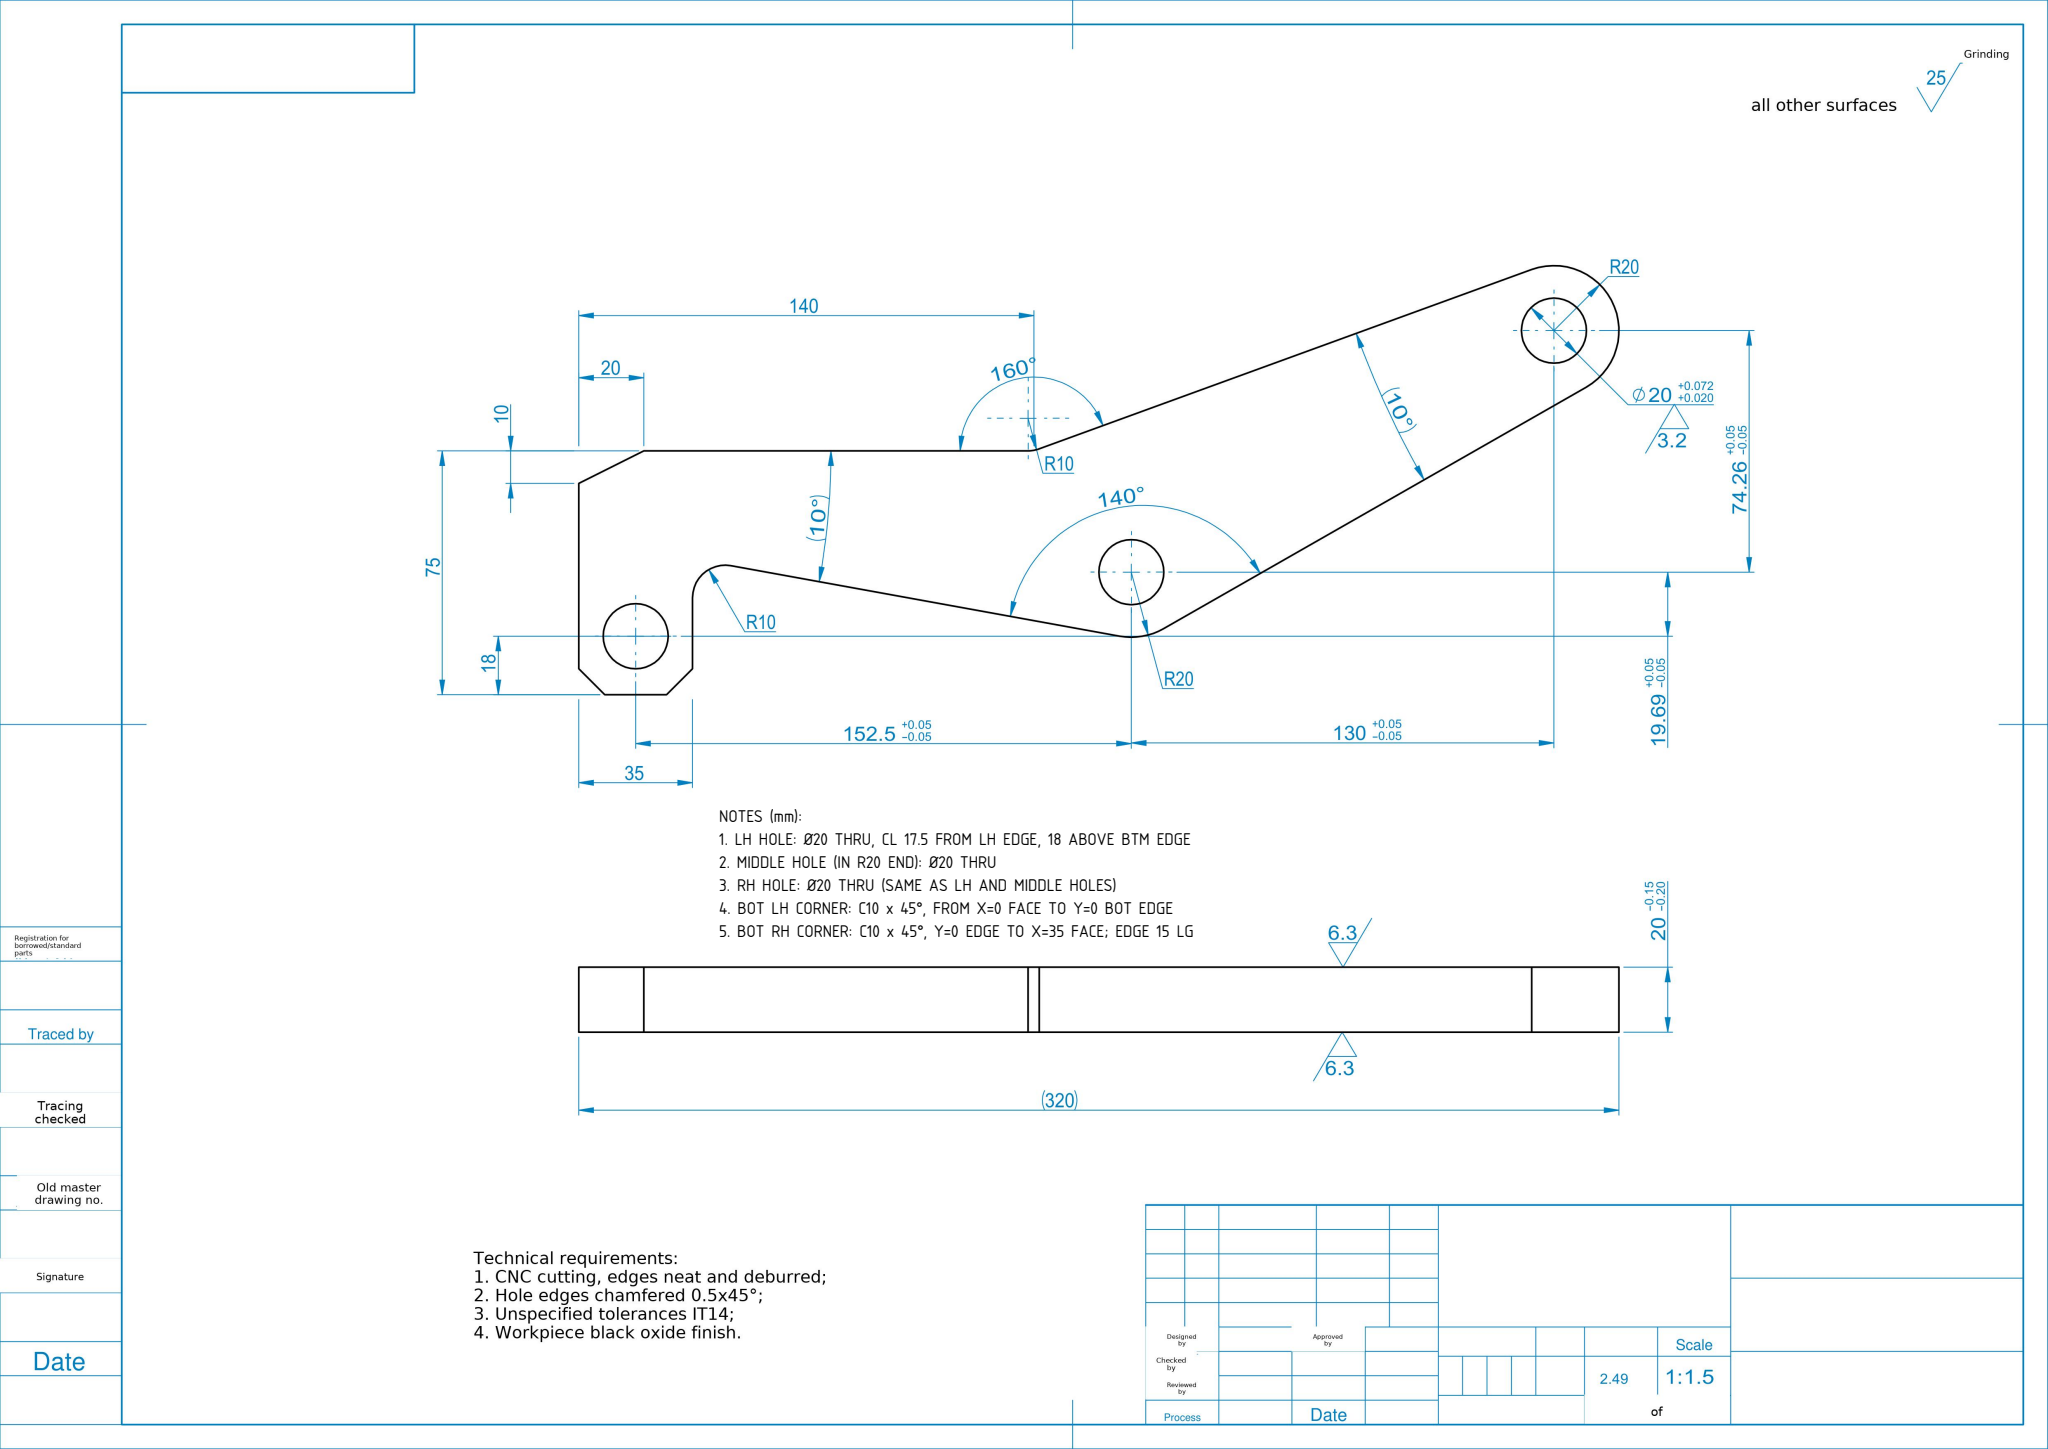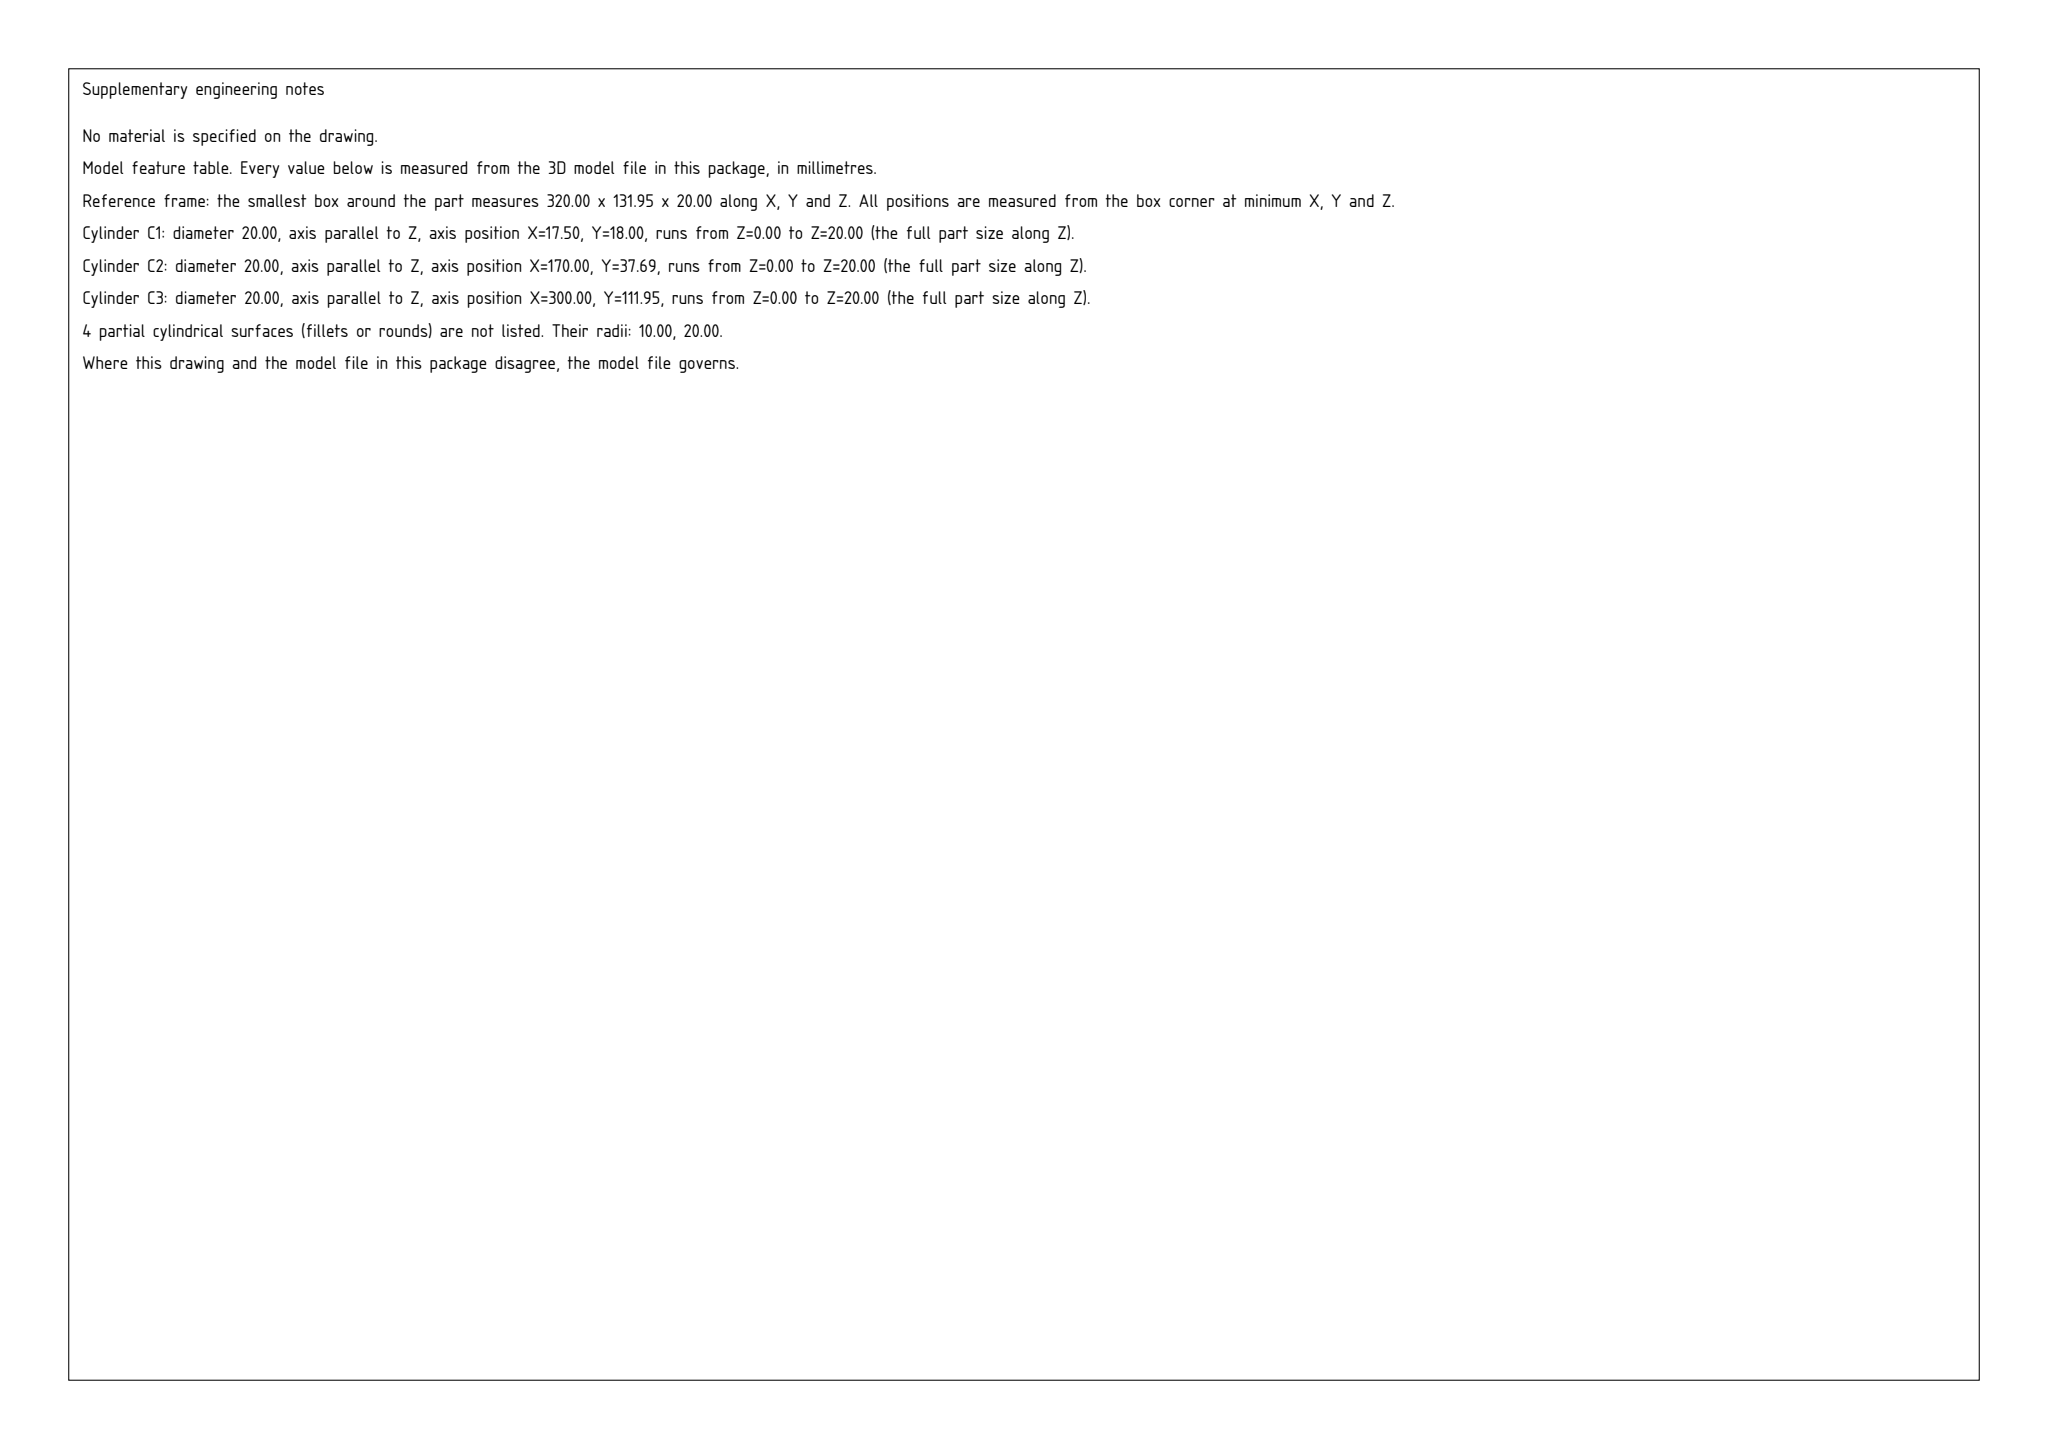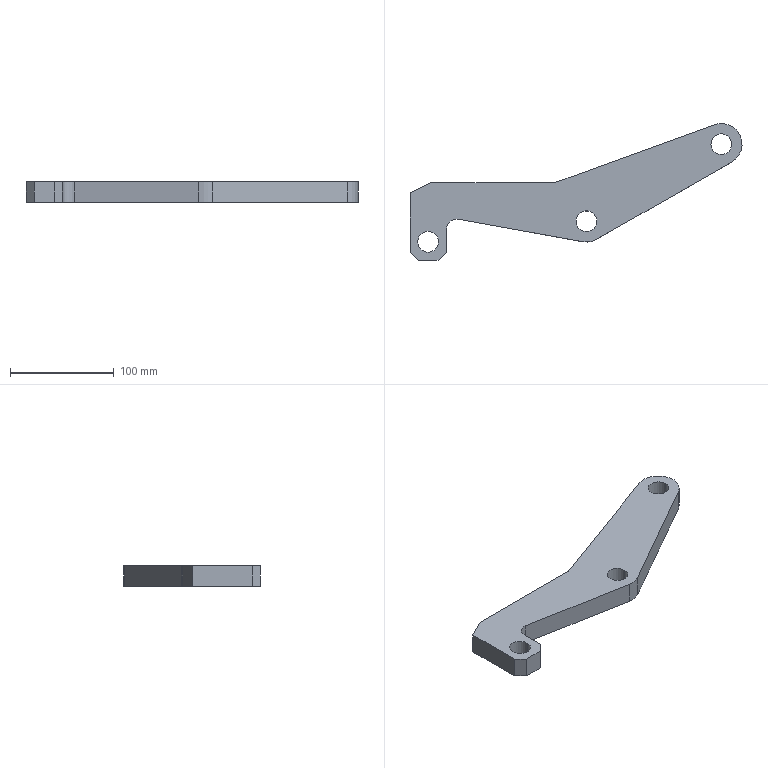Part | SolidWorks | mm | 1 solid | 22 faces | box 320 x 131.95 x 20 mm | volume 319656 mm3 | plane 12 | cylinder 10 | commonest cylinder face diameters 20 x8 40 x2
Drawing notes:
LH HOLE: Ø20 THRU, CL 17.5 FROM LH EDGE, 18 ABOVE BTM EDGE | from the solid: cylinder dia 20.0, axis z, pos (17.5, 18.0), length 20.0 (thru 20 thk)
MIDDLE HOLE (IN R20 END): Ø20 THRU | from the solid: cylinder dia 20.0, axis z, pos (170.0, 37.69), length 20.0, coaxial with 40.0 dia R20 end
RH HOLE: Ø20 THRU (SAME AS LH AND MIDDLE HOLES) | from the solid: cylinder dia 20.0, axis z, pos (300.0, 111.95), coaxial with 40.0 dia R20 end
BOT LH CORNER: C10 x 45°, FROM X=0 FACE TO Y=0 BOT EDGE | from the solid: Planes x=0, y=0 of left block (bbox min corner); chamfer face runs 45° between them, legs 10 x 10, i.e. starts 10 up x=0 face and 10 along y=0 edge
BOT RH CORNER: C10 x 45°, Y=0 EDGE TO X=35 FACE; EDGE 15 LG | from the solid: Planes y=0 and x=35; 45° chamfer legs 10 x 10 -> bottom edge runs x=10 to x=25 (15 lg), x=35 face starts at y=10
build123d program:
from build123d import *

# Parameters (mm, degrees)
BOSS_EXTRUDE1_DEPTH = 10
SKETCH2_R           = 10
CUT_EXTRUDE1_DEPTH  = 347.715
CHAMFER2_SIZE       = 8
CHAMFER3_SIZE       = 20
CHAMFER3_SIZE2      = 10
FILLET1_R           = 10
SKETCH5_R           = 10
CUT_EXTRUDE3_DEPTH  = 347.715
SKETCH7_R           = 10
CUT_EXTRUDE5_DEPTH  = 347.715
CUT_EXTRUDE6_DEPTH  = 347.715
FILLET4_R           = 10


with BuildPart() as part:
    # Sketch1 → Boss-Extrude1 (new, symmetric)
    with BuildSketch(Plane.XY):
        with BuildLine():
            Line((140, 75), (293.16, 130.746))
            ThreePointArc((293.16, 130.746), (318.146, 120.362), (309.92, 94.585))
            Line((309.92, 94.585), (179.92, 20.325))
            ThreePointArc((179.92, 20.325), (173.382, 17.979), (166.436, 18.011))
            Line((166.436, 18.011), (45, 40))
            Line((45, 40), (35, 30))
            Line((35, 30), (35, 0))
            Line((35, 0), (0, 0))
            Line((0, 0), (0, 75))
            Line((0, 75), (140, 75))
        make_face()
    extrude(amount=BOSS_EXTRUDE1_DEPTH, both=True)

    # Sketch2 → Cut-Extrude1 (cut, through all)
    with BuildSketch(Plane.XY.offset(10)):
        with Locations((300, 111.952)):
            Circle(SKETCH2_R)
    extrude(amount=-CUT_EXTRUDE1_DEPTH, mode=Mode.SUBTRACT)

    # Chamfer2
    chamfer2_edges = [part.edges().sort_by_distance(p)[0] for p in [
        (35, 0, 0),
        (0, 0, 0),
    ]]
    chamfer(chamfer2_edges, length=CHAMFER2_SIZE)

    # Chamfer3
    chamfer3_edges = [part.edges().sort_by_distance(p)[0] for p in [
        (0, 75, 0),
    ]]
    chamfer3_side = [part.faces().sort_by_distance(p)[0] for p in [
        (70, 75, 0),
    ]]
    chamfer(chamfer3_edges, length=CHAMFER3_SIZE, length2=CHAMFER3_SIZE2, reference=chamfer3_side[0])

    # Fillet1
    fillet1_edges = [part.edges().sort_by_distance(p)[0] for p in [
        (140, 75, 0),
    ]]
    fillet(fillet1_edges, radius=FILLET1_R)

    # Sketch5 → Cut-Extrude3 (cut, through all)
    with BuildSketch(Plane.XY.offset(10)):
        with Locations((17.5, 18)):
            Circle(SKETCH5_R)
    extrude(amount=-CUT_EXTRUDE3_DEPTH, mode=Mode.SUBTRACT)

    # Sketch7 → Cut-Extrude5 (cut, through all)
    with BuildSketch(Plane.XY.offset(10)):
        with Locations((170, 37.691)):
            Circle(SKETCH7_R)
    extrude(amount=-CUT_EXTRUDE5_DEPTH, mode=Mode.SUBTRACT)

    # Sketch8 → Cut-Extrude6 (cut, through all)
    with BuildSketch(Plane.XY.offset(10)):
        Polygon((35, 30), (35, 41.811), (45, 40), align=None)
    extrude(amount=-CUT_EXTRUDE6_DEPTH, mode=Mode.SUBTRACT)

    # Fillet4
    fillet4_edges = [part.edges().sort_by_distance(p)[0] for p in [
        (35, 41.811, 0),
    ]]
    fillet(fillet4_edges, radius=FILLET4_R)


solid = part.part
STEP:
#1=CARTESIAN_POINT('',(160.,37.691,-10.));
#2=VERTEX_POINT('',#1);
#3=CARTESIAN_POINT('',(180.,37.691,-10.));
#4=VERTEX_POINT('',#3);
#5=CARTESIAN_POINT('',(170.,37.691,-10.));
#6=DIRECTION('',(0.,0.,1.));
#7=DIRECTION('',(1.,0.,0.));
#8=AXIS2_PLACEMENT_3D('',#5,#6,#7);
#9=CIRCLE('',#8,10.);
#10=EDGE_CURVE('',#2,#4,#9,.T.);
#11=ORIENTED_EDGE('',*,*,#10,.F.);
#12=CARTESIAN_POINT('',(160.,37.691,10.));
#13=VERTEX_POINT('',#12);
#14=CARTESIAN_POINT('',(160.,37.691,-10.));
#15=DIRECTION('',(0.,0.,1.));
#16=VECTOR('',#15,1000.);
#17=LINE('',#14,#16);
#18=EDGE_CURVE('',#2,#13,#17,.T.);
#19=ORIENTED_EDGE('',*,*,#18,.T.);
#20=CARTESIAN_POINT('',(180.,37.691,10.));
#21=VERTEX_POINT('',#20);
#22=CARTESIAN_POINT('',(170.,37.691,10.));
#23=DIRECTION('',(0.,0.,1.));
#24=DIRECTION('',(1.,0.,0.));
#25=AXIS2_PLACEMENT_3D('',#22,#23,#24);
#26=CIRCLE('',#25,10.);
#27=EDGE_CURVE('',#13,#21,#26,.T.);
#28=ORIENTED_EDGE('',*,*,#27,.T.);
#29=CARTESIAN_POINT('',(180.,37.691,-10.));
#30=DIRECTION('',(0.,0.,1.));
#31=VECTOR('',#30,1000.);
#32=LINE('',#29,#31);
#33=EDGE_CURVE('',#4,#21,#32,.T.);
#34=ORIENTED_EDGE('',*,*,#33,.F.);
#35=EDGE_LOOP('',(#11,#19,#28,#34));
#36=FACE_OUTER_BOUND('',#35,.T.);
#37=CARTESIAN_POINT('',(170.,37.691,-10.));
#38=DIRECTION('',(0.,0.,1.));
#39=DIRECTION('',(1.,0.,0.));
#40=AXIS2_PLACEMENT_3D('',#37,#38,#39);
#41=CYLINDRICAL_SURFACE('',#40,10.);
#42=ADVANCED_FACE('',(#36),#41,.F.);
#43=CARTESIAN_POINT('',(7.5,18.,-10.));
#44=VERTEX_POINT('',#43);
#45=CARTESIAN_POINT('',(27.5,18.,-10.));
#46=VERTEX_POINT('',#45);
#47=CARTESIAN_POINT('',(17.5,18.,-10.));
#48=DIRECTION('',(0.,0.,1.));
#49=DIRECTION('',(1.,0.,0.));
#50=AXIS2_PLACEMENT_3D('',#47,#48,#49);
#51=CIRCLE('',#50,10.);
#52=EDGE_CURVE('',#44,#46,#51,.T.);
#53=ORIENTED_EDGE('',*,*,#52,.F.);
#54=CARTESIAN_POINT('',(7.5,18.,10.));
#55=VERTEX_POINT('',#54);
#56=CARTESIAN_POINT('',(7.5,18.,-10.));
#57=DIRECTION('',(0.,0.,1.));
#58=VECTOR('',#57,1000.);
#59=LINE('',#56,#58);
#60=EDGE_CURVE('',#44,#55,#59,.T.);
#61=ORIENTED_EDGE('',*,*,#60,.T.);
#62=CARTESIAN_POINT('',(27.5,18.,10.));
#63=VERTEX_POINT('',#62);
#64=CARTESIAN_POINT('',(17.5,18.,10.));
#65=DIRECTION('',(0.,0.,1.));
#66=DIRECTION('',(1.,0.,0.));
#67=AXIS2_PLACEMENT_3D('',#64,#65,#66);
#68=CIRCLE('',#67,10.);
#69=EDGE_CURVE('',#55,#63,#68,.T.);
#70=ORIENTED_EDGE('',*,*,#69,.T.);
#71=CARTESIAN_POINT('',(27.5,18.,-10.));
#72=DIRECTION('',(0.,0.,1.));
#73=VECTOR('',#72,1000.);
#74=LINE('',#71,#73);
#75=EDGE_CURVE('',#46,#63,#74,.T.);
#76=ORIENTED_EDGE('',*,*,#75,.F.);
#77=EDGE_LOOP('',(#53,#61,#70,#76));
#78=FACE_OUTER_BOUND('',#77,.T.);
#79=CARTESIAN_POINT('',(17.5,18.,-10.));
#80=DIRECTION('',(0.,0.,1.));
#81=DIRECTION('',(1.,0.,0.));
#82=AXIS2_PLACEMENT_3D('',#79,#80,#81);
#83=CYLINDRICAL_SURFACE('',#82,10.);
#84=ADVANCED_FACE('',(#78),#83,.F.);
#85=CARTESIAN_POINT('',(290.,111.952,-10.));
#86=VERTEX_POINT('',#85);
#87=CARTESIAN_POINT('',(310.,111.952,-10.));
#88=VERTEX_POINT('',#87);
#89=CARTESIAN_POINT('',(300.,111.952,-10.));
#90=DIRECTION('',(0.,0.,1.));
#91=DIRECTION('',(1.,0.,0.));
#92=AXIS2_PLACEMENT_3D('',#89,#90,#91);
#93=CIRCLE('',#92,10.);
#94=EDGE_CURVE('',#86,#88,#93,.T.);
#95=ORIENTED_EDGE('',*,*,#94,.F.);
#96=CARTESIAN_POINT('',(290.,111.952,10.));
#97=VERTEX_POINT('',#96);
#98=CARTESIAN_POINT('',(290.,111.952,-10.));
#99=DIRECTION('',(0.,0.,1.));
#100=VECTOR('',#99,1000.);
#101=LINE('',#98,#100);
#102=EDGE_CURVE('',#86,#97,#101,.T.);
#103=ORIENTED_EDGE('',*,*,#102,.T.);
#104=CARTESIAN_POINT('',(310.,111.952,10.));
#105=VERTEX_POINT('',#104);
#106=CARTESIAN_POINT('',(300.,111.952,10.));
#107=DIRECTION('',(0.,0.,1.));
#108=DIRECTION('',(1.,0.,0.));
#109=AXIS2_PLACEMENT_3D('',#106,#107,#108);
#110=CIRCLE('',#109,10.);
#111=EDGE_CURVE('',#97,#105,#110,.T.);
#112=ORIENTED_EDGE('',*,*,#111,.T.);
#113=CARTESIAN_POINT('',(310.,111.952,-10.));
#114=DIRECTION('',(0.,0.,1.));
#115=VECTOR('',#114,1000.);
#116=LINE('',#113,#115);
#117=EDGE_CURVE('',#88,#105,#116,.T.);
#118=ORIENTED_EDGE('',*,*,#117,.F.);
#119=EDGE_LOOP('',(#95,#103,#112,#118));
#120=FACE_OUTER_BOUND('',#119,.T.);
#121=CARTESIAN_POINT('',(300.,111.952,-10.));
#122=DIRECTION('',(0.,0.,1.));
#123=DIRECTION('',(1.,0.,0.));
#124=AXIS2_PLACEMENT_3D('',#121,#122,#123);
#125=CYLINDRICAL_SURFACE('',#124,10.);
#126=ADVANCED_FACE('',(#120),#125,.F.);
#127=CARTESIAN_POINT('',(46.782,39.677,10.));
#128=VERTEX_POINT('',#127);
#129=CARTESIAN_POINT('',(166.436,18.011,10.));
#130=VERTEX_POINT('',#129);
#131=CARTESIAN_POINT('',(45.,40.,10.));
#132=DIRECTION('',(0.984,-0.1782,0.));
#133=VECTOR('',#132,1000.);
#134=LINE('',#131,#133);
#135=EDGE_CURVE('',#128,#130,#134,.T.);
#136=ORIENTED_EDGE('',*,*,#135,.F.);
#137=CARTESIAN_POINT('',(46.782,39.677,-10.));
#138=VERTEX_POINT('',#137);
#139=CARTESIAN_POINT('',(46.782,39.677,-10.));
#140=DIRECTION('',(0.,0.,-1.));
#141=VECTOR('',#140,1000.);
#142=LINE('',#139,#141);
#143=EDGE_CURVE('',#128,#138,#142,.T.);
#144=ORIENTED_EDGE('',*,*,#143,.T.);
#145=CARTESIAN_POINT('',(166.436,18.011,-10.));
#146=VERTEX_POINT('',#145);
#147=CARTESIAN_POINT('',(45.,40.,-10.));
#148=DIRECTION('',(0.984,-0.1782,0.));
#149=VECTOR('',#148,1000.);
#150=LINE('',#147,#149);
#151=EDGE_CURVE('',#138,#146,#150,.T.);
#152=ORIENTED_EDGE('',*,*,#151,.T.);
#153=CARTESIAN_POINT('',(166.436,18.011,10.));
#154=DIRECTION('',(0.,0.,-1.));
#155=VECTOR('',#154,1000.);
#156=LINE('',#153,#155);
#157=EDGE_CURVE('',#130,#146,#156,.T.);
#158=ORIENTED_EDGE('',*,*,#157,.F.);
#159=EDGE_LOOP('',(#136,#144,#152,#158));
#160=FACE_OUTER_BOUND('',#159,.T.);
#161=CARTESIAN_POINT('',(45.,40.,10.));
#162=DIRECTION('',(0.1782,0.984,0.));
#163=DIRECTION('',(-0.984,0.1782,0.));
#164=AXIS2_PLACEMENT_3D('',#161,#162,#163);
#165=PLANE('',#164);
#166=ADVANCED_FACE('',(#160),#165,.F.);
#167=CARTESIAN_POINT('',(179.92,20.325,-10.));
#168=VERTEX_POINT('',#167);
#169=CARTESIAN_POINT('',(170.,37.691,-10.));
#170=DIRECTION('',(0.,0.,1.));
#171=DIRECTION('',(1.,0.,0.));
#172=AXIS2_PLACEMENT_3D('',#169,#170,#171);
#173=CIRCLE('',#172,20.);
#174=EDGE_CURVE('',#146,#168,#173,.T.);
#175=ORIENTED_EDGE('',*,*,#174,.T.);
#176=CARTESIAN_POINT('',(179.92,20.325,10.));
#177=VERTEX_POINT('',#176);
#178=CARTESIAN_POINT('',(179.92,20.325,10.));
#179=DIRECTION('',(0.,0.,-1.));
#180=VECTOR('',#179,1000.);
#181=LINE('',#178,#180);
#182=EDGE_CURVE('',#177,#168,#181,.T.);
#183=ORIENTED_EDGE('',*,*,#182,.F.);
#184=CARTESIAN_POINT('',(170.,37.691,10.));
#185=DIRECTION('',(0.,0.,1.));
#186=DIRECTION('',(1.,0.,0.));
#187=AXIS2_PLACEMENT_3D('',#184,#185,#186);
#188=CIRCLE('',#187,20.);
#189=EDGE_CURVE('',#130,#177,#188,.T.);
#190=ORIENTED_EDGE('',*,*,#189,.F.);
#191=ORIENTED_EDGE('',*,*,#157,.T.);
#192=EDGE_LOOP('',(#175,#183,#190,#191));
#193=FACE_OUTER_BOUND('',#192,.T.);
#194=CARTESIAN_POINT('',(170.,37.691,10.));
#195=DIRECTION('',(0.,0.,-1.));
#196=DIRECTION('',(-1.,0.,0.));
#197=AXIS2_PLACEMENT_3D('',#194,#195,#196);
#198=CYLINDRICAL_SURFACE('',#197,20.);
#199=ADVANCED_FACE('',(#193),#198,.T.);
#200=CARTESIAN_POINT('',(309.92,94.585,-10.));
#201=VERTEX_POINT('',#200);
#202=CARTESIAN_POINT('',(179.92,20.325,-10.));
#203=DIRECTION('',(0.8683,0.496,0.));
#204=VECTOR('',#203,1000.);
#205=LINE('',#202,#204);
#206=EDGE_CURVE('',#168,#201,#205,.T.);
#207=ORIENTED_EDGE('',*,*,#206,.T.);
#208=CARTESIAN_POINT('',(309.92,94.585,10.));
#209=VERTEX_POINT('',#208);
#210=CARTESIAN_POINT('',(309.92,94.585,10.));
#211=DIRECTION('',(0.,0.,-1.));
#212=VECTOR('',#211,1000.);
#213=LINE('',#210,#212);
#214=EDGE_CURVE('',#209,#201,#213,.T.);
#215=ORIENTED_EDGE('',*,*,#214,.F.);
#216=CARTESIAN_POINT('',(179.92,20.325,10.));
#217=DIRECTION('',(0.8683,0.496,0.));
#218=VECTOR('',#217,1000.);
#219=LINE('',#216,#218);
#220=EDGE_CURVE('',#177,#209,#219,.T.);
#221=ORIENTED_EDGE('',*,*,#220,.F.);
#222=ORIENTED_EDGE('',*,*,#182,.T.);
#223=EDGE_LOOP('',(#207,#215,#221,#222));
#224=FACE_OUTER_BOUND('',#223,.T.);
#225=CARTESIAN_POINT('',(179.92,20.325,10.));
#226=DIRECTION('',(-0.496,0.8683,0.));
#227=DIRECTION('',(-0.8683,-0.496,0.));
#228=AXIS2_PLACEMENT_3D('',#225,#226,#227);
#229=PLANE('',#228);
#230=ADVANCED_FACE('',(#224),#229,.F.);
#231=CARTESIAN_POINT('',(293.16,130.746,-10.));
#232=VERTEX_POINT('',#231);
#233=CARTESIAN_POINT('',(300.,111.952,-10.));
#234=DIRECTION('',(0.,0.,1.));
#235=DIRECTION('',(1.,0.,0.));
#236=AXIS2_PLACEMENT_3D('',#233,#234,#235);
#237=CIRCLE('',#236,20.);
#238=EDGE_CURVE('',#201,#232,#237,.T.);
#239=ORIENTED_EDGE('',*,*,#238,.T.);
#240=CARTESIAN_POINT('',(293.16,130.746,10.));
#241=VERTEX_POINT('',#240);
#242=CARTESIAN_POINT('',(293.16,130.746,10.));
#243=DIRECTION('',(0.,0.,-1.));
#244=VECTOR('',#243,1000.);
#245=LINE('',#242,#244);
#246=EDGE_CURVE('',#241,#232,#245,.T.);
#247=ORIENTED_EDGE('',*,*,#246,.F.);
#248=CARTESIAN_POINT('',(300.,111.952,10.));
#249=DIRECTION('',(0.,0.,1.));
#250=DIRECTION('',(1.,0.,0.));
#251=AXIS2_PLACEMENT_3D('',#248,#249,#250);
#252=CIRCLE('',#251,20.);
#253=EDGE_CURVE('',#209,#241,#252,.T.);
#254=ORIENTED_EDGE('',*,*,#253,.F.);
#255=ORIENTED_EDGE('',*,*,#214,.T.);
#256=EDGE_LOOP('',(#239,#247,#254,#255));
#257=FACE_OUTER_BOUND('',#256,.T.);
#258=CARTESIAN_POINT('',(300.,111.952,10.));
#259=DIRECTION('',(0.,0.,-1.));
#260=DIRECTION('',(-1.,0.,0.));
#261=AXIS2_PLACEMENT_3D('',#258,#259,#260);
#262=CYLINDRICAL_SURFACE('',#261,20.);
#263=ADVANCED_FACE('',(#257),#262,.T.);
#264=CARTESIAN_POINT('',(141.657,75.603,-10.));
#265=VERTEX_POINT('',#264);
#266=CARTESIAN_POINT('',(140.,75.,-10.));
#267=DIRECTION('',(-0.9397,-0.342,0.));
#268=VECTOR('',#267,1000.);
#269=LINE('',#266,#268);
#270=EDGE_CURVE('',#232,#265,#269,.T.);
#271=ORIENTED_EDGE('',*,*,#270,.T.);
#272=CARTESIAN_POINT('',(141.657,75.603,10.));
#273=VERTEX_POINT('',#272);
#274=CARTESIAN_POINT('',(141.657,75.603,10.));
#275=DIRECTION('',(0.,0.,1.));
#276=VECTOR('',#275,1000.);
#277=LINE('',#274,#276);
#278=EDGE_CURVE('',#265,#273,#277,.T.);
#279=ORIENTED_EDGE('',*,*,#278,.T.);
#280=CARTESIAN_POINT('',(140.,75.,10.));
#281=DIRECTION('',(-0.9397,-0.342,0.));
#282=VECTOR('',#281,1000.);
#283=LINE('',#280,#282);
#284=EDGE_CURVE('',#241,#273,#283,.T.);
#285=ORIENTED_EDGE('',*,*,#284,.F.);
#286=ORIENTED_EDGE('',*,*,#246,.T.);
#287=EDGE_LOOP('',(#271,#279,#285,#286));
#288=FACE_OUTER_BOUND('',#287,.T.);
#289=CARTESIAN_POINT('',(140.,75.,10.));
#290=DIRECTION('',(0.342,-0.9397,0.));
#291=DIRECTION('',(0.9397,0.342,0.));
#292=AXIS2_PLACEMENT_3D('',#289,#290,#291);
#293=PLANE('',#292);
#294=ADVANCED_FACE('',(#288),#293,.F.);
#295=CARTESIAN_POINT('',(138.237,75.,10.));
#296=VERTEX_POINT('',#295);
#297=CARTESIAN_POINT('',(20.,75.,10.));
#298=VERTEX_POINT('',#297);
#299=CARTESIAN_POINT('',(0.,75.,10.));
#300=DIRECTION('',(-1.,-0.,0.));
#301=VECTOR('',#300,1000.);
#302=LINE('',#299,#301);
#303=EDGE_CURVE('',#296,#298,#302,.T.);
#304=ORIENTED_EDGE('',*,*,#303,.F.);
#305=CARTESIAN_POINT('',(138.237,75.,-10.));
#306=VERTEX_POINT('',#305);
#307=CARTESIAN_POINT('',(138.237,75.,-10.));
#308=DIRECTION('',(0.,0.,-1.));
#309=VECTOR('',#308,1000.);
#310=LINE('',#307,#309);
#311=EDGE_CURVE('',#296,#306,#310,.T.);
#312=ORIENTED_EDGE('',*,*,#311,.T.);
#313=CARTESIAN_POINT('',(20.,75.,-10.));
#314=VERTEX_POINT('',#313);
#315=CARTESIAN_POINT('',(0.,75.,-10.));
#316=DIRECTION('',(-1.,-0.,0.));
#317=VECTOR('',#316,1000.);
#318=LINE('',#315,#317);
#319=EDGE_CURVE('',#306,#314,#318,.T.);
#320=ORIENTED_EDGE('',*,*,#319,.T.);
#321=CARTESIAN_POINT('',(20.,75.,10.));
#322=DIRECTION('',(0.,0.,1.));
#323=VECTOR('',#322,1000.);
#324=LINE('',#321,#323);
#325=EDGE_CURVE('',#314,#298,#324,.T.);
#326=ORIENTED_EDGE('',*,*,#325,.T.);
#327=EDGE_LOOP('',(#304,#312,#320,#326));
#328=FACE_OUTER_BOUND('',#327,.T.);
#329=CARTESIAN_POINT('',(0.,75.,10.));
#330=DIRECTION('',(0.,-1.,0.));
#331=DIRECTION('',(1.,0.,0.));
#332=AXIS2_PLACEMENT_3D('',#329,#330,#331);
#333=PLANE('',#332);
#334=ADVANCED_FACE('',(#328),#333,.F.);
#335=CARTESIAN_POINT('',(-0.,65.,10.));
#336=VERTEX_POINT('',#335);
#337=CARTESIAN_POINT('',(-0.,8.,10.));
#338=VERTEX_POINT('',#337);
#339=CARTESIAN_POINT('',(0.,0.,10.));
#340=DIRECTION('',(0.,-1.,0.));
#341=VECTOR('',#340,1000.);
#342=LINE('',#339,#341);
#343=EDGE_CURVE('',#336,#338,#342,.T.);
#344=ORIENTED_EDGE('',*,*,#343,.F.);
#345=CARTESIAN_POINT('',(-0.,65.,-10.));
#346=VERTEX_POINT('',#345);
#347=CARTESIAN_POINT('',(0.,65.,10.));
#348=DIRECTION('',(0.,0.,-1.));
#349=VECTOR('',#348,1000.);
#350=LINE('',#347,#349);
#351=EDGE_CURVE('',#336,#346,#350,.T.);
#352=ORIENTED_EDGE('',*,*,#351,.T.);
#353=CARTESIAN_POINT('',(0.,8.,-10.));
#354=VERTEX_POINT('',#353);
#355=CARTESIAN_POINT('',(0.,0.,-10.));
#356=DIRECTION('',(0.,-1.,0.));
#357=VECTOR('',#356,1000.);
#358=LINE('',#355,#357);
#359=EDGE_CURVE('',#346,#354,#358,.T.);
#360=ORIENTED_EDGE('',*,*,#359,.T.);
#361=CARTESIAN_POINT('',(0.,8.,10.));
#362=DIRECTION('',(0.,0.,1.));
#363=VECTOR('',#362,1000.);
#364=LINE('',#361,#363);
#365=EDGE_CURVE('',#354,#338,#364,.T.);
#366=ORIENTED_EDGE('',*,*,#365,.T.);
#367=EDGE_LOOP('',(#344,#352,#360,#366));
#368=FACE_OUTER_BOUND('',#367,.T.);
#369=CARTESIAN_POINT('',(0.,0.,10.));
#370=DIRECTION('',(1.,0.,0.));
#371=DIRECTION('',(0.,0.,-1.));
#372=AXIS2_PLACEMENT_3D('',#369,#370,#371);
#373=PLANE('',#372);
#374=ADVANCED_FACE('',(#368),#373,.F.);
#375=CARTESIAN_POINT('',(8.,-0.,-10.));
#376=VERTEX_POINT('',#375);
#377=CARTESIAN_POINT('',(27.,0.,-10.));
#378=VERTEX_POINT('',#377);
#379=CARTESIAN_POINT('',(35.,0.,-10.));
#380=DIRECTION('',(1.,0.,0.));
#381=VECTOR('',#380,1000.);
#382=LINE('',#379,#381);
#383=EDGE_CURVE('',#376,#378,#382,.T.);
#384=ORIENTED_EDGE('',*,*,#383,.T.);
#385=CARTESIAN_POINT('',(27.,-0.,10.));
#386=VERTEX_POINT('',#385);
#387=CARTESIAN_POINT('',(27.,0.,10.));
#388=DIRECTION('',(0.,0.,1.));
#389=VECTOR('',#388,1000.);
#390=LINE('',#387,#389);
#391=EDGE_CURVE('',#378,#386,#390,.T.);
#392=ORIENTED_EDGE('',*,*,#391,.T.);
#393=CARTESIAN_POINT('',(8.,0.,10.));
#394=VERTEX_POINT('',#393);
#395=CARTESIAN_POINT('',(35.,0.,10.));
#396=DIRECTION('',(1.,0.,0.));
#397=VECTOR('',#396,1000.);
#398=LINE('',#395,#397);
#399=EDGE_CURVE('',#394,#386,#398,.T.);
#400=ORIENTED_EDGE('',*,*,#399,.F.);
#401=CARTESIAN_POINT('',(8.,0.,10.));
#402=DIRECTION('',(0.,0.,-1.));
#403=VECTOR('',#402,1000.);
#404=LINE('',#401,#403);
#405=EDGE_CURVE('',#394,#376,#404,.T.);
#406=ORIENTED_EDGE('',*,*,#405,.T.);
#407=EDGE_LOOP('',(#384,#392,#400,#406));
#408=FACE_OUTER_BOUND('',#407,.T.);
#409=CARTESIAN_POINT('',(35.,0.,10.));
#410=DIRECTION('',(-0.,1.,0.));
#411=DIRECTION('',(-1.,-0.,0.));
#412=AXIS2_PLACEMENT_3D('',#409,#410,#411);
#413=PLANE('',#412);
#414=ADVANCED_FACE('',(#408),#413,.F.);
#415=CARTESIAN_POINT('',(35.,8.,-10.));
#416=VERTEX_POINT('',#415);
#417=CARTESIAN_POINT('',(35.,29.837,-10.));
#418=VERTEX_POINT('',#417);
#419=CARTESIAN_POINT('',(35.,30.,-10.));
#420=DIRECTION('',(0.,1.,0.));
#421=VECTOR('',#420,1000.);
#422=LINE('',#419,#421);
#423=EDGE_CURVE('',#416,#418,#422,.T.);
#424=ORIENTED_EDGE('',*,*,#423,.T.);
#425=CARTESIAN_POINT('',(35.,29.837,10.));
#426=VERTEX_POINT('',#425);
#427=CARTESIAN_POINT('',(35.,29.837,10.));
#428=DIRECTION('',(0.,0.,1.));
#429=VECTOR('',#428,1000.);
#430=LINE('',#427,#429);
#431=EDGE_CURVE('',#418,#426,#430,.T.);
#432=ORIENTED_EDGE('',*,*,#431,.T.);
#433=CARTESIAN_POINT('',(35.,8.,10.));
#434=VERTEX_POINT('',#433);
#435=CARTESIAN_POINT('',(35.,30.,10.));
#436=DIRECTION('',(0.,1.,0.));
#437=VECTOR('',#436,1000.);
#438=LINE('',#435,#437);
#439=EDGE_CURVE('',#434,#426,#438,.T.);
#440=ORIENTED_EDGE('',*,*,#439,.F.);
#441=CARTESIAN_POINT('',(35.,8.,10.));
#442=DIRECTION('',(0.,0.,-1.));
#443=VECTOR('',#442,1000.);
#444=LINE('',#441,#443);
#445=EDGE_CURVE('',#434,#416,#444,.T.);
#446=ORIENTED_EDGE('',*,*,#445,.T.);
#447=EDGE_LOOP('',(#424,#432,#440,#446));
#448=FACE_OUTER_BOUND('',#447,.T.);
#449=CARTESIAN_POINT('',(35.,30.,10.));
#450=DIRECTION('',(-1.,0.,0.));
#451=DIRECTION('',(0.,0.,1.));
#452=AXIS2_PLACEMENT_3D('',#449,#450,#451);
#453=PLANE('',#452);
#454=ADVANCED_FACE('',(#448),#453,.F.);
#455=ORIENTED_EDGE('',*,*,#439,.T.);
#456=CARTESIAN_POINT('',(45.,29.837,10.));
#457=DIRECTION('',(0.,0.,-1.));
#458=DIRECTION('',(1.,-0.,0.));
#459=AXIS2_PLACEMENT_3D('',#456,#457,#458);
#460=CIRCLE('',#459,10.);
#461=EDGE_CURVE('',#426,#128,#460,.T.);
#462=ORIENTED_EDGE('',*,*,#461,.T.);
#463=ORIENTED_EDGE('',*,*,#135,.T.);
#464=ORIENTED_EDGE('',*,*,#189,.T.);
#465=ORIENTED_EDGE('',*,*,#220,.T.);
#466=ORIENTED_EDGE('',*,*,#253,.T.);
#467=ORIENTED_EDGE('',*,*,#284,.T.);
#468=CARTESIAN_POINT('',(138.237,85.,10.));
#469=DIRECTION('',(0.,0.,-1.));
#470=DIRECTION('',(1.,-0.,0.));
#471=AXIS2_PLACEMENT_3D('',#468,#469,#470);
#472=CIRCLE('',#471,10.);
#473=EDGE_CURVE('',#273,#296,#472,.T.);
#474=ORIENTED_EDGE('',*,*,#473,.T.);
#475=ORIENTED_EDGE('',*,*,#303,.T.);
#476=CARTESIAN_POINT('',(125.076,127.538,10.));
#477=DIRECTION('',(-0.8944,-0.4472,0.));
#478=VECTOR('',#477,1000.);
#479=LINE('',#476,#478);
#480=EDGE_CURVE('',#298,#336,#479,.T.);
#481=ORIENTED_EDGE('',*,*,#480,.T.);
#482=ORIENTED_EDGE('',*,*,#343,.T.);
#483=CARTESIAN_POINT('',(70.154,-62.154,10.));
#484=DIRECTION('',(0.7071,-0.7071,0.));
#485=VECTOR('',#484,1000.);
#486=LINE('',#483,#485);
#487=EDGE_CURVE('',#338,#394,#486,.T.);
#488=ORIENTED_EDGE('',*,*,#487,.T.);
#489=ORIENTED_EDGE('',*,*,#399,.T.);
#490=CARTESIAN_POINT('',(117.346,90.346,10.));
#491=DIRECTION('',(0.7071,0.7071,0.));
#492=VECTOR('',#491,1000.);
#493=LINE('',#490,#492);
#494=EDGE_CURVE('',#386,#434,#493,.T.);
#495=ORIENTED_EDGE('',*,*,#494,.T.);
#496=EDGE_LOOP('',(#455,#462,#463,#464,#465,#466,#467,#474,#475,#481,#482,#488,#489,#495));
#497=FACE_OUTER_BOUND('',#496,.T.);
#498=CARTESIAN_POINT('',(170.,37.691,10.));
#499=DIRECTION('',(0.,0.,1.));
#500=DIRECTION('',(1.,0.,0.));
#501=AXIS2_PLACEMENT_3D('',#498,#499,#500);
#502=CIRCLE('',#501,10.);
#503=EDGE_CURVE('',#21,#13,#502,.T.);
#504=ORIENTED_EDGE('',*,*,#503,.F.);
#505=ORIENTED_EDGE('',*,*,#27,.F.);
#506=EDGE_LOOP('',(#504,#505));
#507=FACE_BOUND('',#506,.T.);
#508=CARTESIAN_POINT('',(17.5,18.,10.));
#509=DIRECTION('',(0.,0.,1.));
#510=DIRECTION('',(1.,0.,0.));
#511=AXIS2_PLACEMENT_3D('',#508,#509,#510);
#512=CIRCLE('',#511,10.);
#513=EDGE_CURVE('',#63,#55,#512,.T.);
#514=ORIENTED_EDGE('',*,*,#513,.F.);
#515=ORIENTED_EDGE('',*,*,#69,.F.);
#516=EDGE_LOOP('',(#514,#515));
#517=FACE_BOUND('',#516,.T.);
#518=CARTESIAN_POINT('',(300.,111.952,10.));
#519=DIRECTION('',(0.,0.,1.));
#520=DIRECTION('',(1.,0.,0.));
#521=AXIS2_PLACEMENT_3D('',#518,#519,#520);
#522=CIRCLE('',#521,10.);
#523=EDGE_CURVE('',#105,#97,#522,.T.);
#524=ORIENTED_EDGE('',*,*,#523,.F.);
#525=ORIENTED_EDGE('',*,*,#111,.F.);
#526=EDGE_LOOP('',(#524,#525));
#527=FACE_BOUND('',#526,.T.);
#528=CARTESIAN_POINT('',(170.,37.691,10.));
#529=DIRECTION('',(0.,0.,1.));
#530=DIRECTION('',(1.,0.,0.));
#531=AXIS2_PLACEMENT_3D('',#528,#529,#530);
#532=PLANE('',#531);
#533=ADVANCED_FACE('',(#497,#507,#517,#527),#532,.T.);
#534=CARTESIAN_POINT('',(170.,37.691,-10.));
#535=DIRECTION('',(0.,0.,1.));
#536=DIRECTION('',(1.,0.,0.));
#537=AXIS2_PLACEMENT_3D('',#534,#535,#536);
#538=CIRCLE('',#537,10.);
#539=EDGE_CURVE('',#4,#2,#538,.T.);
#540=ORIENTED_EDGE('',*,*,#539,.T.);
#541=ORIENTED_EDGE('',*,*,#10,.T.);
#542=EDGE_LOOP('',(#540,#541));
#543=FACE_BOUND('',#542,.T.);
#544=CARTESIAN_POINT('',(17.5,18.,-10.));
#545=DIRECTION('',(0.,0.,1.));
#546=DIRECTION('',(1.,0.,0.));
#547=AXIS2_PLACEMENT_3D('',#544,#545,#546);
#548=CIRCLE('',#547,10.);
#549=EDGE_CURVE('',#46,#44,#548,.T.);
#550=ORIENTED_EDGE('',*,*,#549,.T.);
#551=ORIENTED_EDGE('',*,*,#52,.T.);
#552=EDGE_LOOP('',(#550,#551));
#553=FACE_BOUND('',#552,.T.);
#554=CARTESIAN_POINT('',(300.,111.952,-10.));
#555=DIRECTION('',(0.,0.,1.));
#556=DIRECTION('',(1.,0.,0.));
#557=AXIS2_PLACEMENT_3D('',#554,#555,#556);
#558=CIRCLE('',#557,10.);
#559=EDGE_CURVE('',#88,#86,#558,.T.);
#560=ORIENTED_EDGE('',*,*,#559,.T.);
#561=ORIENTED_EDGE('',*,*,#94,.T.);
#562=EDGE_LOOP('',(#560,#561));
#563=FACE_BOUND('',#562,.T.);
#564=ORIENTED_EDGE('',*,*,#151,.F.);
#565=CARTESIAN_POINT('',(45.,29.837,-10.));
#566=DIRECTION('',(0.,0.,1.));
#567=DIRECTION('',(1.,0.,0.));
#568=AXIS2_PLACEMENT_3D('',#565,#566,#567);
#569=CIRCLE('',#568,10.);
#570=EDGE_CURVE('',#138,#418,#569,.T.);
#571=ORIENTED_EDGE('',*,*,#570,.T.);
#572=ORIENTED_EDGE('',*,*,#423,.F.);
#573=CARTESIAN_POINT('',(35.,8.,-10.));
#574=DIRECTION('',(-0.7071,-0.7071,0.));
#575=VECTOR('',#574,1000.);
#576=LINE('',#573,#575);
#577=EDGE_CURVE('',#416,#378,#576,.T.);
#578=ORIENTED_EDGE('',*,*,#577,.T.);
#579=ORIENTED_EDGE('',*,*,#383,.F.);
#580=CARTESIAN_POINT('',(8.,0.,-10.));
#581=DIRECTION('',(-0.7071,0.7071,0.));
#582=VECTOR('',#581,1000.);
#583=LINE('',#580,#582);
#584=EDGE_CURVE('',#376,#354,#583,.T.);
#585=ORIENTED_EDGE('',*,*,#584,.T.);
#586=ORIENTED_EDGE('',*,*,#359,.F.);
#587=CARTESIAN_POINT('',(0.,65.,-10.));
#588=DIRECTION('',(0.8944,0.4472,0.));
#589=VECTOR('',#588,1000.);
#590=LINE('',#587,#589);
#591=EDGE_CURVE('',#346,#314,#590,.T.);
#592=ORIENTED_EDGE('',*,*,#591,.T.);
#593=ORIENTED_EDGE('',*,*,#319,.F.);
#594=CARTESIAN_POINT('',(138.237,85.,-10.));
#595=DIRECTION('',(0.,0.,1.));
#596=DIRECTION('',(1.,0.,0.));
#597=AXIS2_PLACEMENT_3D('',#594,#595,#596);
#598=CIRCLE('',#597,10.);
#599=EDGE_CURVE('',#306,#265,#598,.T.);
#600=ORIENTED_EDGE('',*,*,#599,.T.);
#601=ORIENTED_EDGE('',*,*,#270,.F.);
#602=ORIENTED_EDGE('',*,*,#238,.F.);
#603=ORIENTED_EDGE('',*,*,#206,.F.);
#604=ORIENTED_EDGE('',*,*,#174,.F.);
#605=EDGE_LOOP('',(#564,#571,#572,#578,#579,#585,#586,#592,#593,#600,#601,#602,#603,#604));
#606=FACE_OUTER_BOUND('',#605,.T.);
#607=CARTESIAN_POINT('',(170.,37.691,-10.));
#608=DIRECTION('',(0.,0.,1.));
#609=DIRECTION('',(1.,0.,0.));
#610=AXIS2_PLACEMENT_3D('',#607,#608,#609);
#611=PLANE('',#610);
#612=ADVANCED_FACE('',(#543,#553,#563,#606),#611,.F.);
#613=ORIENTED_EDGE('',*,*,#102,.F.);
#614=ORIENTED_EDGE('',*,*,#559,.F.);
#615=ORIENTED_EDGE('',*,*,#117,.T.);
#616=ORIENTED_EDGE('',*,*,#523,.T.);
#617=EDGE_LOOP('',(#613,#614,#615,#616));
#618=FACE_OUTER_BOUND('',#617,.T.);
#619=CARTESIAN_POINT('',(300.,111.952,-10.));
#620=DIRECTION('',(0.,0.,1.));
#621=DIRECTION('',(1.,0.,0.));
#622=AXIS2_PLACEMENT_3D('',#619,#620,#621);
#623=CYLINDRICAL_SURFACE('',#622,10.);
#624=ADVANCED_FACE('',(#618),#623,.F.);
#625=ORIENTED_EDGE('',*,*,#494,.F.);
#626=ORIENTED_EDGE('',*,*,#391,.F.);
#627=ORIENTED_EDGE('',*,*,#577,.F.);
#628=ORIENTED_EDGE('',*,*,#445,.F.);
#629=EDGE_LOOP('',(#625,#626,#627,#628));
#630=FACE_OUTER_BOUND('',#629,.T.);
#631=CARTESIAN_POINT('',(35.,8.,10.));
#632=DIRECTION('',(-0.7071,0.7071,0.));
#633=DIRECTION('',(0.,0.,-1.));
#634=AXIS2_PLACEMENT_3D('',#631,#632,#633);
#635=PLANE('',#634);
#636=ADVANCED_FACE('',(#630),#635,.F.);
#637=ORIENTED_EDGE('',*,*,#487,.F.);
#638=ORIENTED_EDGE('',*,*,#365,.F.);
#639=ORIENTED_EDGE('',*,*,#584,.F.);
#640=ORIENTED_EDGE('',*,*,#405,.F.);
#641=EDGE_LOOP('',(#637,#638,#639,#640));
#642=FACE_OUTER_BOUND('',#641,.T.);
#643=CARTESIAN_POINT('',(8.,0.,10.));
#644=DIRECTION('',(0.7071,0.7071,0.));
#645=DIRECTION('',(0.,0.,-1.));
#646=AXIS2_PLACEMENT_3D('',#643,#644,#645);
#647=PLANE('',#646);
#648=ADVANCED_FACE('',(#642),#647,.F.);
#649=ORIENTED_EDGE('',*,*,#480,.F.);
#650=ORIENTED_EDGE('',*,*,#325,.F.);
#651=ORIENTED_EDGE('',*,*,#591,.F.);
#652=ORIENTED_EDGE('',*,*,#351,.F.);
#653=EDGE_LOOP('',(#649,#650,#651,#652));
#654=FACE_OUTER_BOUND('',#653,.T.);
#655=CARTESIAN_POINT('',(0.,65.,10.));
#656=DIRECTION('',(0.4472,-0.8944,0.));
#657=DIRECTION('',(0.,0.,-1.));
#658=AXIS2_PLACEMENT_3D('',#655,#656,#657);
#659=PLANE('',#658);
#660=ADVANCED_FACE('',(#654),#659,.F.);
#661=ORIENTED_EDGE('',*,*,#473,.F.);
#662=ORIENTED_EDGE('',*,*,#278,.F.);
#663=ORIENTED_EDGE('',*,*,#599,.F.);
#664=ORIENTED_EDGE('',*,*,#311,.F.);
#665=EDGE_LOOP('',(#661,#662,#663,#664));
#666=FACE_OUTER_BOUND('',#665,.T.);
#667=CARTESIAN_POINT('',(138.237,85.,10.));
#668=DIRECTION('',(0.,0.,1.));
#669=DIRECTION('',(1.,0.,0.));
#670=AXIS2_PLACEMENT_3D('',#667,#668,#669);
#671=CYLINDRICAL_SURFACE('',#670,10.);
#672=ADVANCED_FACE('',(#666),#671,.F.);
#673=ORIENTED_EDGE('',*,*,#60,.F.);
#674=ORIENTED_EDGE('',*,*,#549,.F.);
#675=ORIENTED_EDGE('',*,*,#75,.T.);
#676=ORIENTED_EDGE('',*,*,#513,.T.);
#677=EDGE_LOOP('',(#673,#674,#675,#676));
#678=FACE_OUTER_BOUND('',#677,.T.);
#679=CARTESIAN_POINT('',(17.5,18.,-10.));
#680=DIRECTION('',(0.,0.,1.));
#681=DIRECTION('',(1.,0.,0.));
#682=AXIS2_PLACEMENT_3D('',#679,#680,#681);
#683=CYLINDRICAL_SURFACE('',#682,10.);
#684=ADVANCED_FACE('',(#678),#683,.F.);
#685=ORIENTED_EDGE('',*,*,#18,.F.);
#686=ORIENTED_EDGE('',*,*,#539,.F.);
#687=ORIENTED_EDGE('',*,*,#33,.T.);
#688=ORIENTED_EDGE('',*,*,#503,.T.);
#689=EDGE_LOOP('',(#685,#686,#687,#688));
#690=FACE_OUTER_BOUND('',#689,.T.);
#691=CARTESIAN_POINT('',(170.,37.691,-10.));
#692=DIRECTION('',(0.,0.,1.));
#693=DIRECTION('',(1.,0.,0.));
#694=AXIS2_PLACEMENT_3D('',#691,#692,#693);
#695=CYLINDRICAL_SURFACE('',#694,10.);
#696=ADVANCED_FACE('',(#690),#695,.F.);
#697=ORIENTED_EDGE('',*,*,#570,.F.);
#698=ORIENTED_EDGE('',*,*,#143,.F.);
#699=ORIENTED_EDGE('',*,*,#461,.F.);
#700=ORIENTED_EDGE('',*,*,#431,.F.);
#701=EDGE_LOOP('',(#697,#698,#699,#700));
#702=FACE_OUTER_BOUND('',#701,.T.);
#703=CARTESIAN_POINT('',(45.,29.837,10.));
#704=DIRECTION('',(0.,0.,-1.));
#705=DIRECTION('',(-1.,0.,0.));
#706=AXIS2_PLACEMENT_3D('',#703,#704,#705);
#707=CYLINDRICAL_SURFACE('',#706,10.);
#708=ADVANCED_FACE('',(#702),#707,.F.);
#709=CLOSED_SHELL('',(#42,#84,#126,#166,#199,#230,#263,#294,#334,#374,#414,#454,#533,#612,#624,#636,#648,#660,#672,#684,#696,#708));
#710=MANIFOLD_SOLID_BREP('',#709);
#711=CARTESIAN_POINT('',(0.,0.,0.));
#712=DIRECTION('',(0.,0.,1.));
#713=DIRECTION('',(1.,0.,0.));
#714=AXIS2_PLACEMENT_3D('',#711,#712,#713);
#715=(LENGTH_UNIT()NAMED_UNIT(*)SI_UNIT(.MILLI.,.METRE.));
#716=UNCERTAINTY_MEASURE_WITH_UNIT(LENGTH_MEASURE(0.00001),#715,'','');
#717=(NAMED_UNIT(*)PLANE_ANGLE_UNIT()SI_UNIT($,.RADIAN.));
#718=(NAMED_UNIT(*)SI_UNIT($,.STERADIAN.)SOLID_ANGLE_UNIT());
#719=(GEOMETRIC_REPRESENTATION_CONTEXT(3)GLOBAL_UNCERTAINTY_ASSIGNED_CONTEXT((#716))GLOBAL_UNIT_ASSIGNED_CONTEXT((#715,#717,#718))REPRESENTATION_CONTEXT('',''));
#720=ADVANCED_BREP_SHAPE_REPRESENTATION('',(#710,#714),#719);